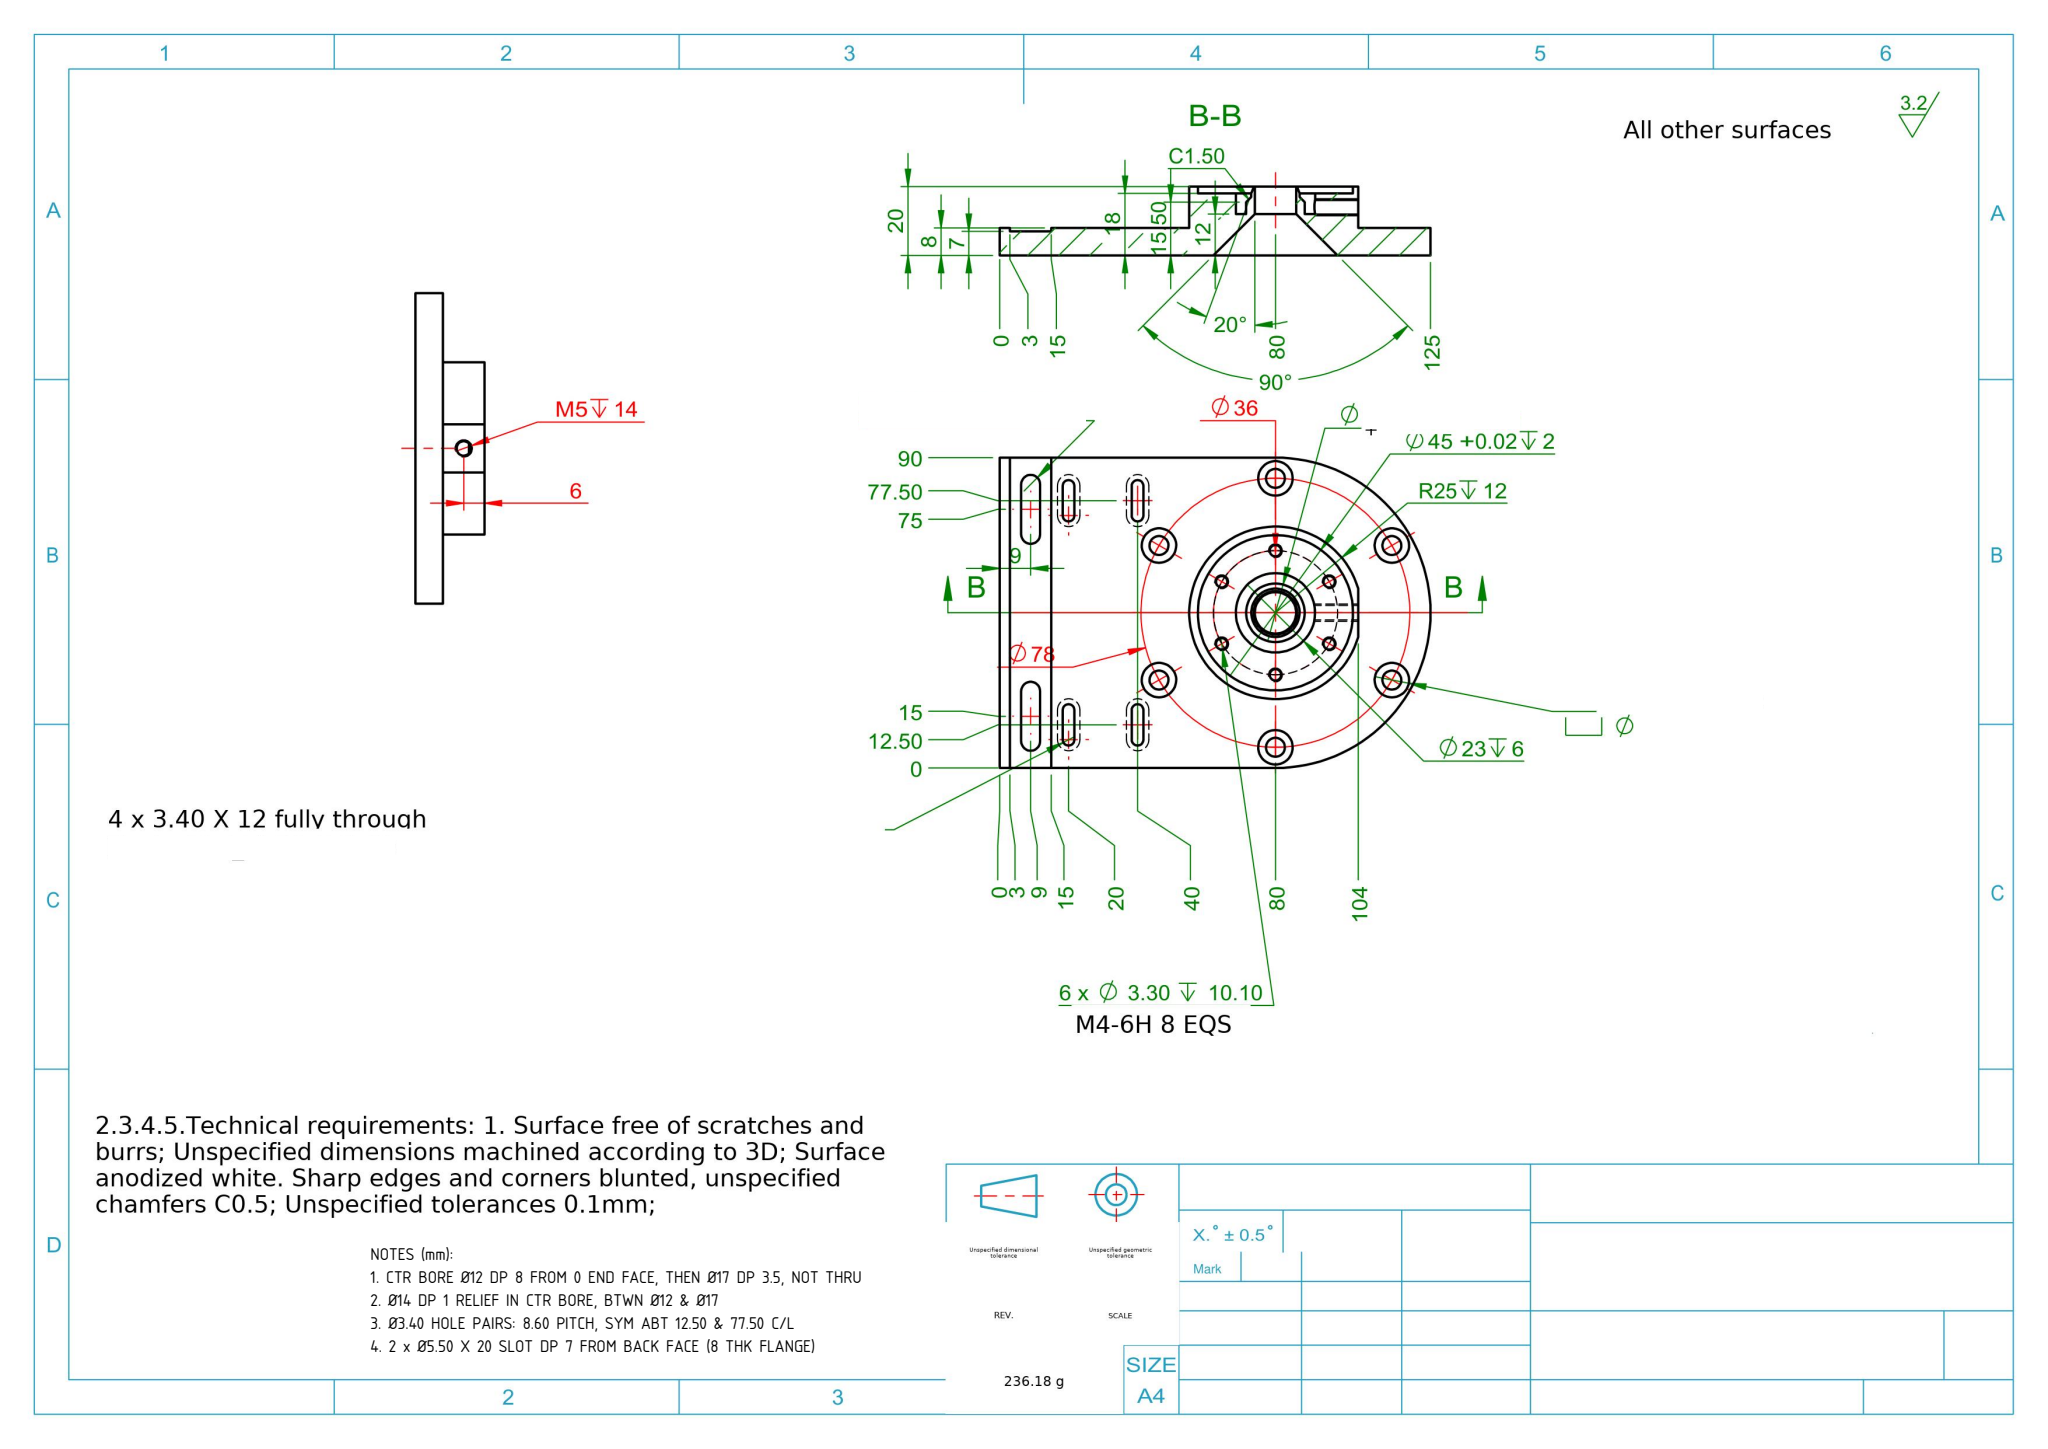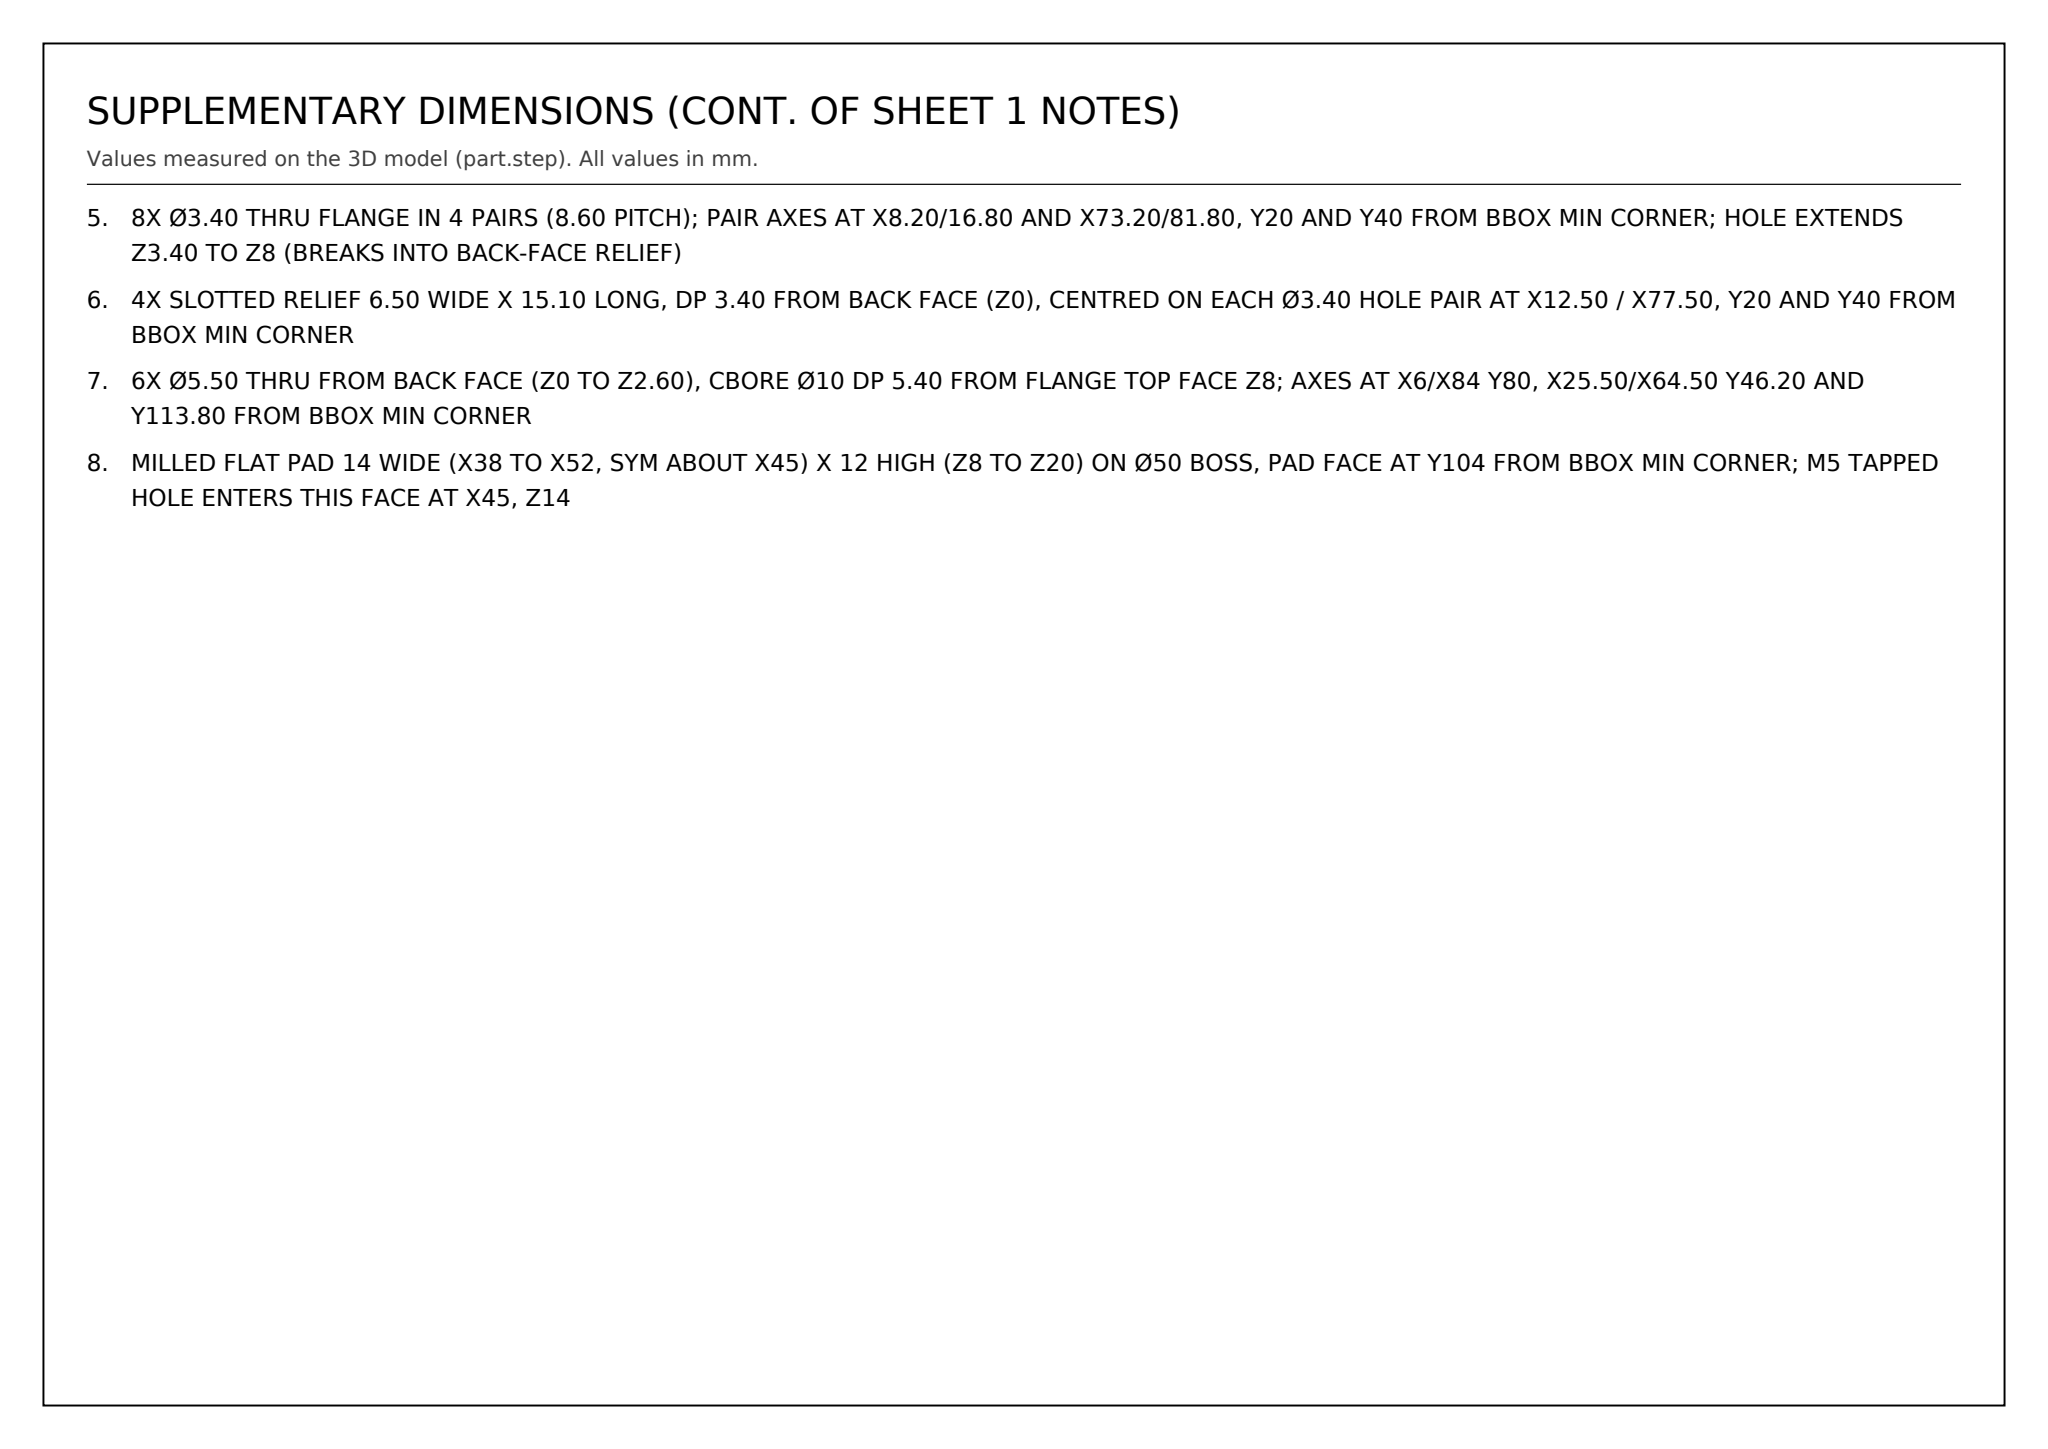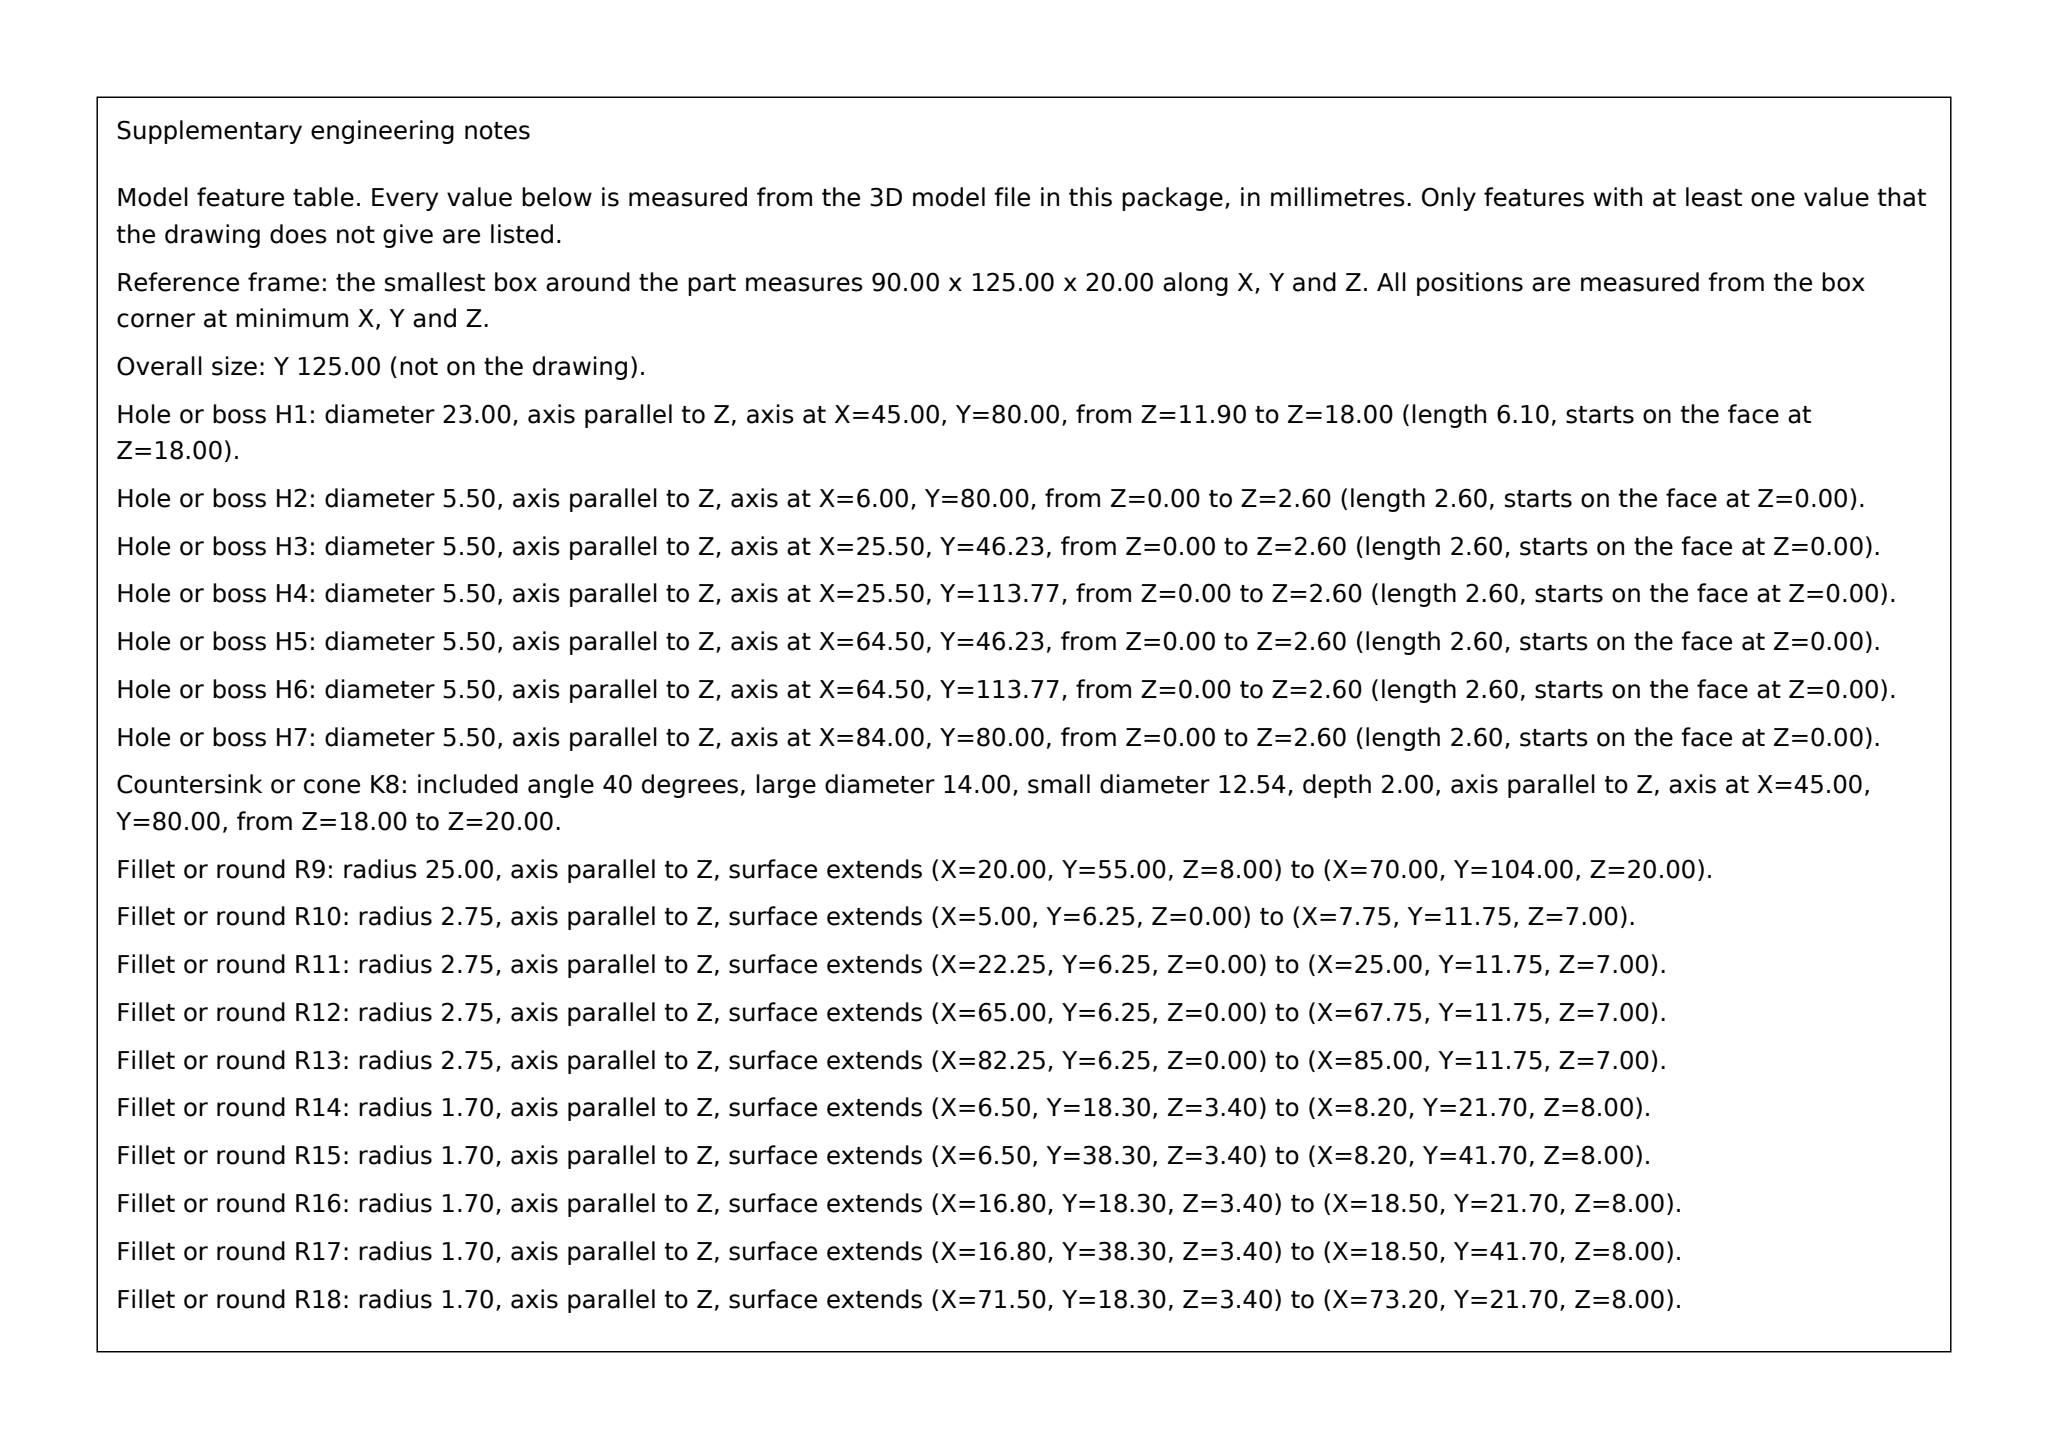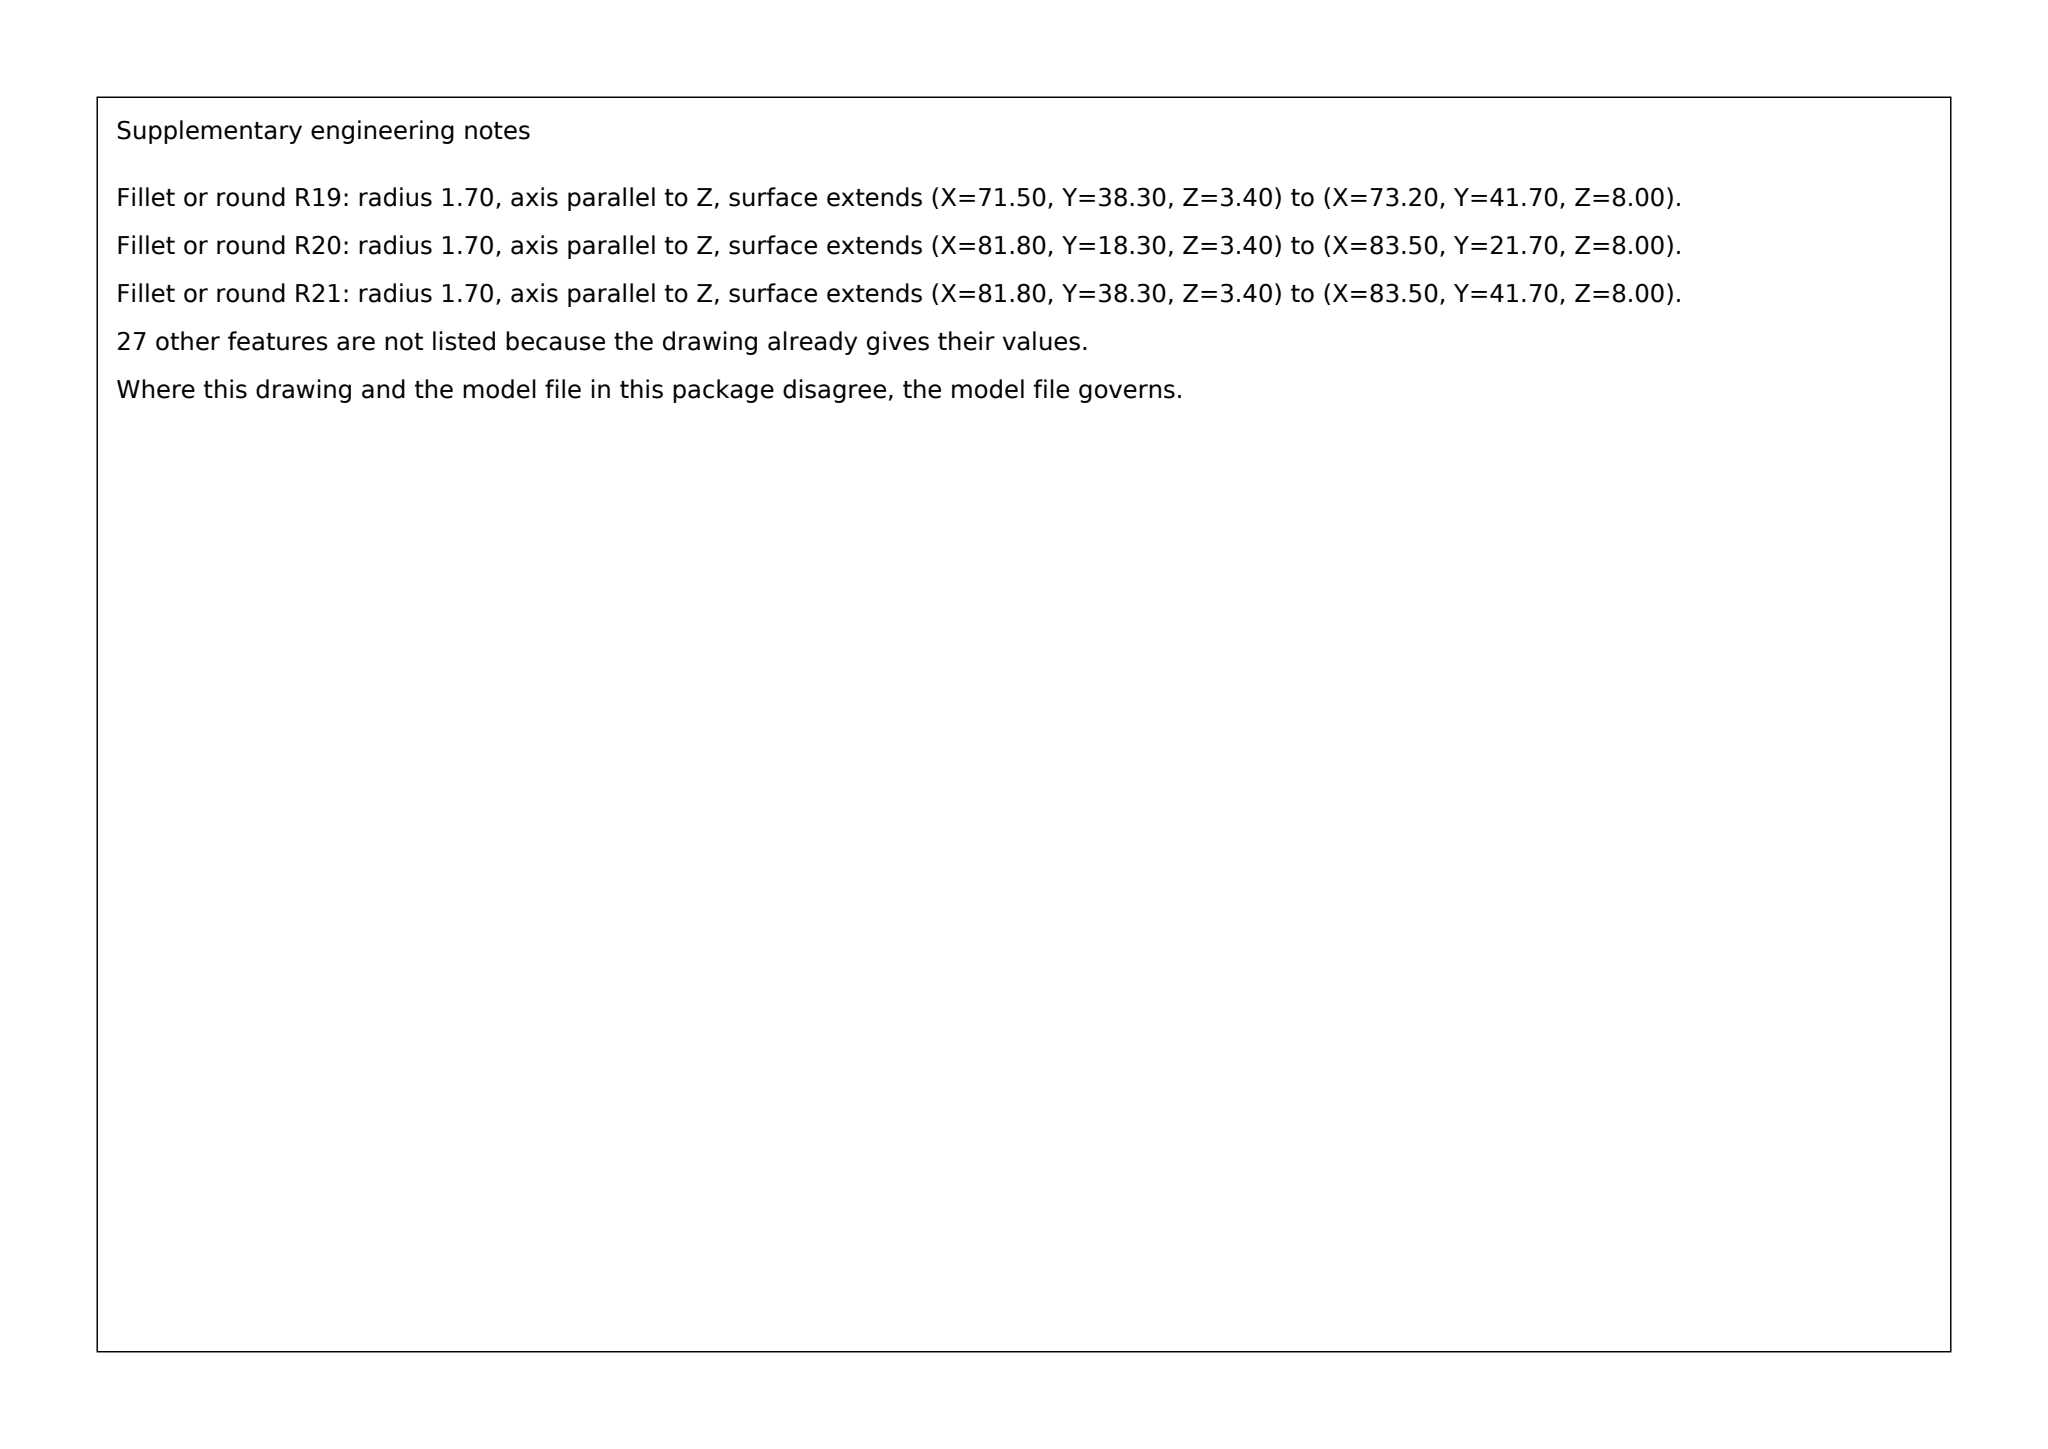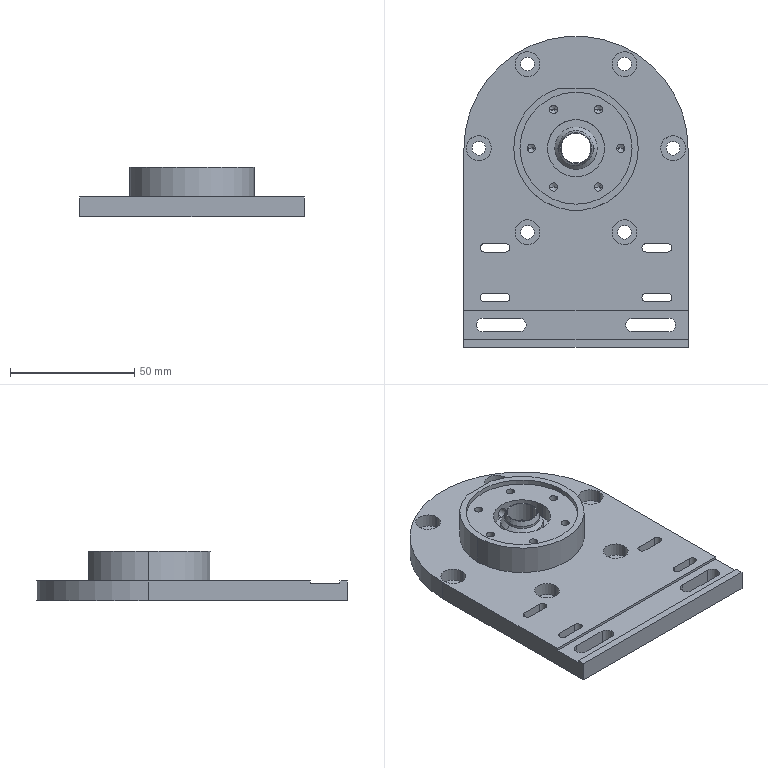Part | SolidWorks | mm | 1 solid | 145 faces | box 90 x 125 x 20 mm | volume 87476 mm3 | cylinder 83 | plane 44 | cone 18 | commonest cylinder face diameters 5.5 x18 6.5 x12 3.4 x12 10 x12 3.3 x12 23 x3 50 x3 17 x2
Drawing notes:
CTR BORE Ø12 DP 8 FROM 0 END FACE, THEN Ø17 DP 3.5, NOT THRU | from the solid: cyl Ø12 z-axis at (45,80) len 8 from z=0; coaxial Ø17 len 3.5 above it, no thru feature
Ø14 DP 1 RELIEF IN CTR BORE, BTWN Ø12 & Ø17 | from the solid: cyl Ø14 z-axis at (45,80) len 1.0, between Ø12 (len 8) and Ø17 (len 3.5)
Ø3.40 HOLE PAIRS: 8.60 PITCH, SYM ABT 12.50 & 77.50 C/L | from the solid: Ø3.4 cylinders at x=8.2 & 16.8 (mean 12.5) and x=73.2 & 81.8 (mean 77.5); 81.8-73.2=16.8-8.2=8.60
2 x Ø5.50 X 20 SLOT DP 7 FROM BACK FACE (8 THK FLANGE) | from the solid: Ø5.5 z-cyls at (7.75,9),(22.25,9),(67.75,9),(82.25,9), len 7.0; flange z-planes 0 and 8; slot ctr dist 14.5 + 5.5 = 20 long
8X Ø3.40 THRU FLANGE IN 4 PAIRS (8.60 PITCH); PAIR AXES AT X8.20/16.80 AND X73.20/81.80, Y20 AND Y40 FROM BBOX MIN CORNER; HOLE EXTENDS Z3.40 TO Z8 (BREAKS INTO BACK-FACE RELIEF) | from the solid: cylinders: 8 x 3.4 dia 180° arcs, axis z at (8.2/16.8/73.2/81.8, y20 & y40), from 3.4 to 8.0
4X SLOTTED RELIEF 6.50 WIDE X 15.10 LONG, DP 3.40 FROM BACK FACE (Z0), CENTRED ON EACH Ø3.40 HOLE PAIR AT X12.50 / X77.50, Y20 AND Y40 FROM BBOX MIN CORNER | from the solid: cylinders: 8 x 6.5 dia 180° arcs, axis z at (8.2/16.8/73.2/81.8, y20 & y40), from 0.0 to 3.4; planes z=3.4 extent x[5.0,20.1] y[16.7,23.3] etc.
6X Ø5.50 THRU FROM BACK FACE (Z0 TO Z2.60), CBORE Ø10 DP 5.40 FROM FLANGE TOP FACE Z8; AXES AT X6/X84 Y80, X25.50/X64.50 Y46.20 AND Y113.80 FROM BBOX MIN CORNER | from the solid: cylinders hole/bore 5.5 z from 0 to 2.6 and hole/bore 10.0 z from 2.6 to 8.0 at [6,80],[84,80],[25.5,46.2],[25.5,113.8],[64.5,46.2],[64.5,113.8]
MILLED FLAT PAD 14 WIDE (X38 TO X52, SYM ABOUT X45) X 12 HIGH (Z8 TO Z20) ON Ø50 BOSS, PAD FACE AT Y104 FROM BBOX MIN CORNER; M5 TAPPED HOLE ENTERS THIS FACE AT X45, Z14 | from the solid: axis_plane normal y, offset 104.0, extent x[38.0,52.0] z[8.0,20.0]; hole/bore 4.2 y-axis at [45,-,14] from 91.3 to 104